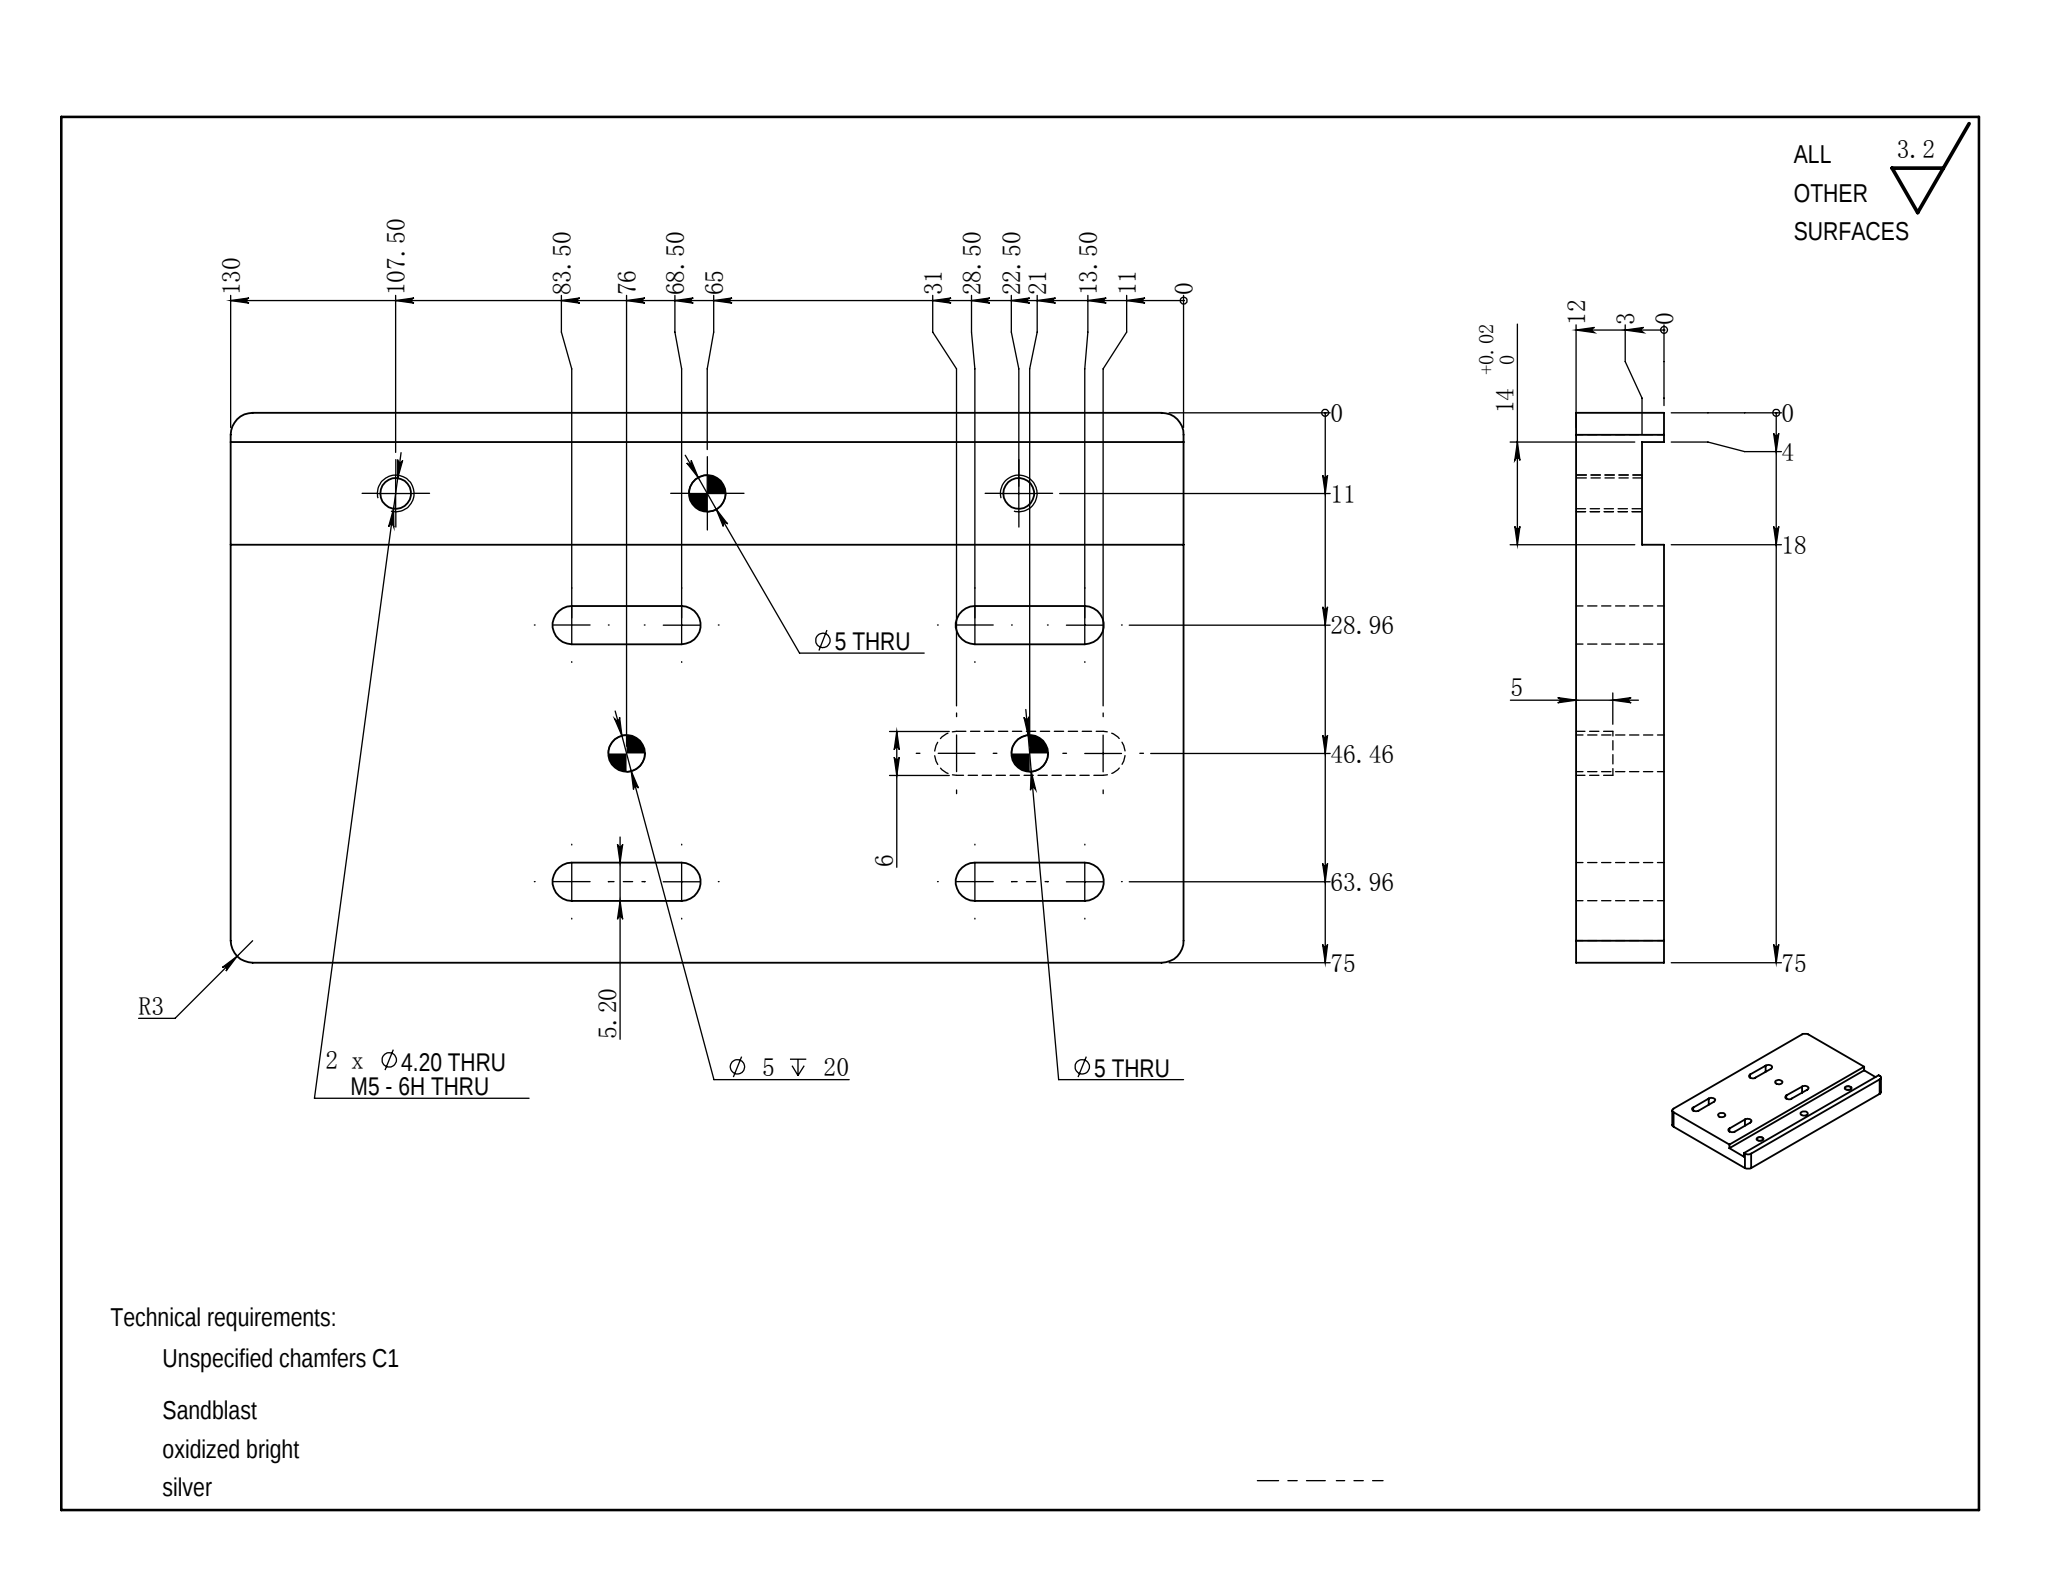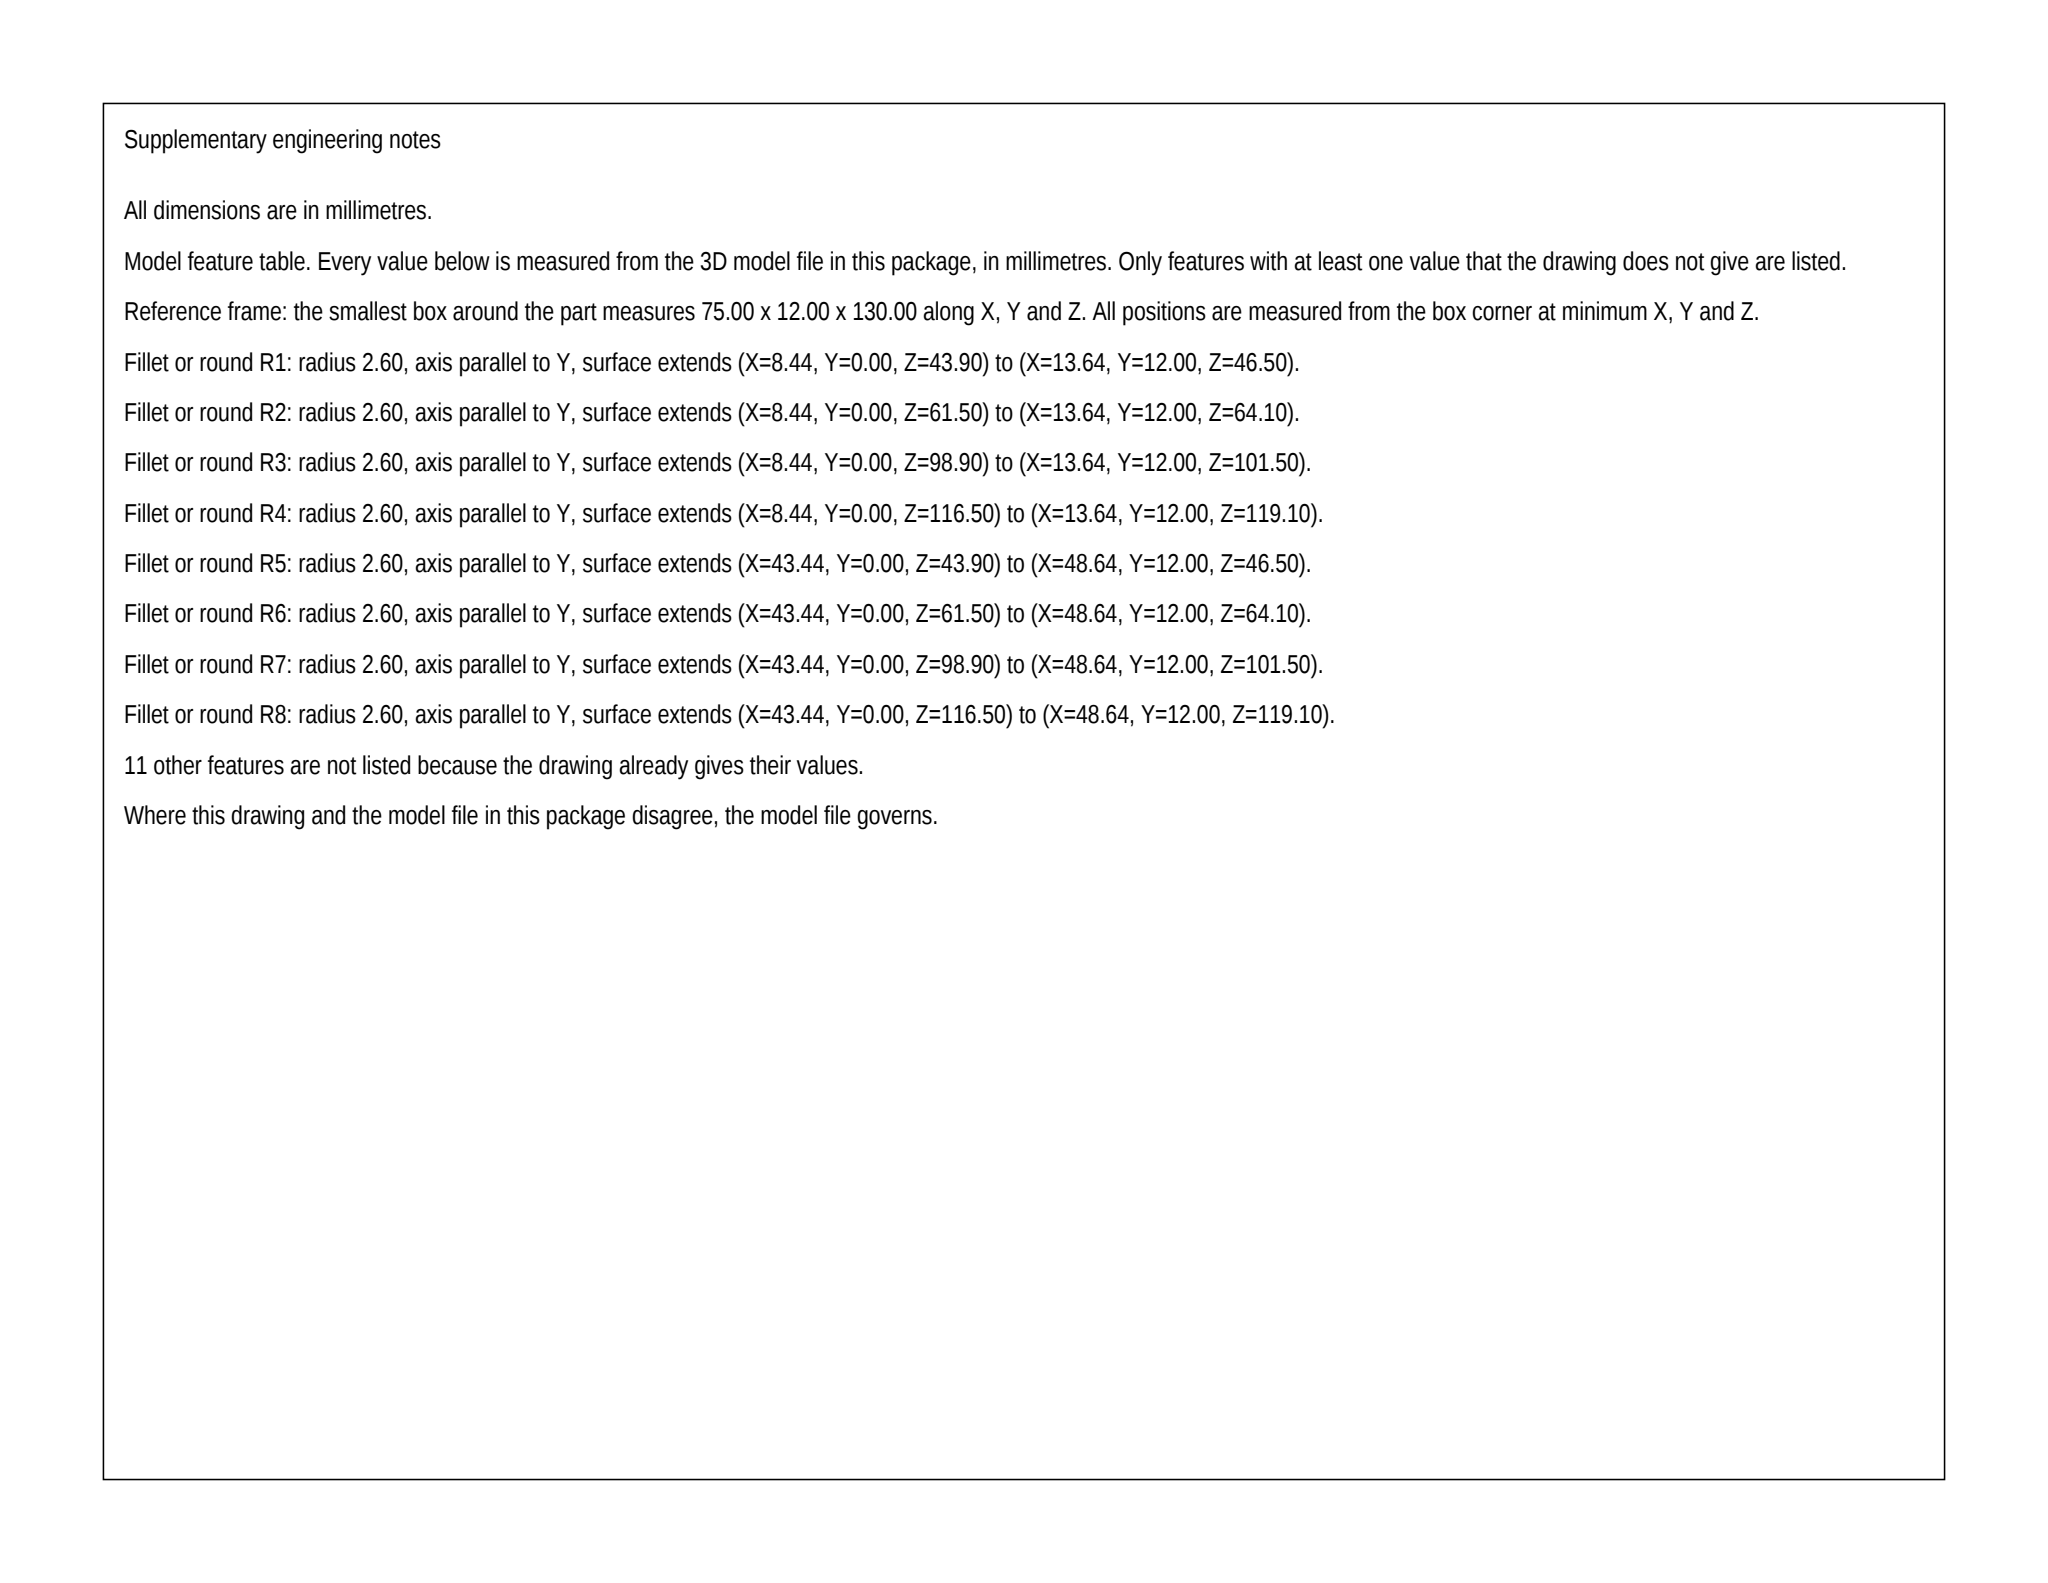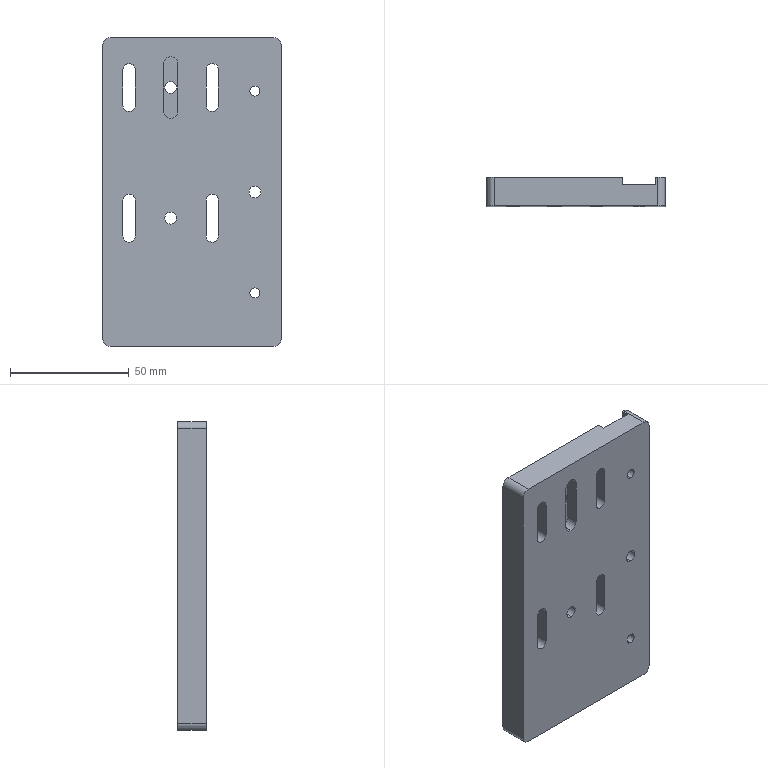Part | SolidWorks | mm | 1 solid | 50 faces | box 75 x 12 x 130 mm | volume 105143 mm3 | cylinder 29 | plane 21 | commonest cylinder face diameters 5.2 x12 6 x7 5 x6 4.2 x4
Drawing notes:
STEP 14 W (4 TO 18) x 3 DP; 9 THK REMAINS | from the solid: x-planes 57 & 71 = Y4/Y18, 14 wide; y-planes 9 & 12 = 3 deep, 9 remaining
4X SLOT 5.20 W x 20.20 LG (15 C-C) THRU 12 | from the solid: Ø5.2 THRU L=12 at x=11.04 & 46.04, z pairs 46.5/61.5 and 101.5/116.5 (15 C-C)
SLOT 6 W x 26 LG (20 C-C) DP 5 W/ Ø5 THRU, CL 46.46 | from the solid: Ø6 L=5 at x=28.54, z=99 & 119 (20 C-C); Ø5 L=7 at x=28.54, z=109; 5+7=12 thk
2X M5 TAP, Ø4.2 DRILL THRU 9 THK, CL 11 AT 22.50 & 107.50 | from the solid: Ø4.2 L=9 at x=64, z=22.5 & 107.5; local thickness 9 at step
Ø5 THRU 9 THK, CL 11 AT 65 | from the solid: Ø5 L=9 at x=64, z=65; local thickness 9 at step
Ø5 THRU 2X AT 46.46 FROM TOP x 76 FROM RIGHT END (NOT ⍋20) | from the solid: cylinder dia 5.0, axis y, pos [28.54, z=54.0], length 12.0 = full 12 plate thickness; 75-28.54=46.46, 130-54=76; count 2
build123d program:
from build123d import *

# Parameters (mm, degrees)
SKETCH1_W                 = 75
SKETCH1_H                 = 130
BOSS_EXTRUDE1_DEPTH       = 12
SKETCH2_W                 = 14
SKETCH2_H                 = 130
CUT_EXTRUDE1_DEPTH        = 3
CUT_EXTRUDE2_DEPTH        = 76.995
LPATTERN1_COUNT           = 2
LPATTERN1_PITCH           = 55
FILLET1_R                 = 3
M5_TAPPED_HOLE1_D         = 4.2
F_5_0_5_DIAMETER_HOLE1_D  = 5
F_5_0_5_DIAMETER_HOLE2_D  = 5
CUT_EXTRUDE3_DEPTH        = 5
SIZE_MM_DOWEL_HOLE1_D     = 5
SIZE_MM_DOWEL_HOLE1_DEPTH = 20
SIZE_MM_DOWEL_HOLE1_TIP   = 1.502


with BuildPart() as part:
    # Sketch1 → Boss-Extrude1 (new body)
    with BuildSketch(Plane(origin=(0, 0, 0), x_dir=(1, 0, 0), z_dir=(0, 1, 0))):
        Rectangle(SKETCH1_W, SKETCH1_H)
    extrude(amount=BOSS_EXTRUDE1_DEPTH)

    # Sketch2 → Cut-Extrude1 (cut)
    with BuildSketch(Plane.XZ.offset(-12)):
        with Locations((26.5, 0)):
            Rectangle(SKETCH2_W, SKETCH2_H)
    extrude(amount=CUT_EXTRUDE1_DEPTH, mode=Mode.SUBTRACT)

    # Sketch3 → Cut-Extrude2 (cut, through all)
    with BuildSketch(Plane(origin=(0, 12, 0), x_dir=(1, 0, 0), z_dir=(0, 1, 0))):
        with BuildLine():
            Line((-29.058, 3.5), (-29.058, 18.5))
            ThreePointArc((-29.058, 18.5), (-26.458, 21.1), (-23.858, 18.5))
            Line((-23.858, 18.5), (-23.858, 3.5))
            ThreePointArc((-23.858, 3.5), (-26.458, 0.9), (-29.058, 3.5))
        make_face()
        with BuildLine():
            Line((11.142, 18.5), (11.142, 3.5))
            ThreePointArc((11.142, 3.5), (8.542, 0.9), (5.942, 3.5))
            Line((5.942, 3.5), (5.942, 18.5))
            ThreePointArc((5.942, 18.5), (8.542, 21.1), (11.142, 18.5))
        make_face()
    cut_extrude2 = extrude(amount=-CUT_EXTRUDE2_DEPTH, mode=Mode.SUBTRACT)

    # LPattern1: Cut-Extrude2 ×2
    with Locations(*[(0, 0, i * LPATTERN1_PITCH) for i in range(1, LPATTERN1_COUNT)]):
        add(cut_extrude2, mode=Mode.SUBTRACT)

    # Fillet1
    fillet1_edges = [part.edges().sort_by_distance(p)[0] for p in [
        (37.5, 6, 65),
        (-37.5, 6, 65),
        (-37.5, 6, -65),
        (37.5, 6, -65),
    ]]
    fillet(fillet1_edges, radius=FILLET1_R)

    # M5 Tapped Hole1 (through all)
    with Locations(Plane(origin=(0, 12, 0), x_dir=(1, 0, 0), z_dir=(0, 1, 0))):
        with Locations((26.5, 42.5), (26.5, -42.5)):
            Hole(M5_TAPPED_HOLE1_D / 2)

    # 5.0 _5_ Diameter Hole1 (through all)
    with Locations(Plane(origin=(0, 9, 0), x_dir=(1, 0, 0), z_dir=(0, 1, 0))):
        with Locations((26.5, 0)):
            Hole(F_5_0_5_DIAMETER_HOLE1_D / 2)

    # 5.0 _5_ Diameter Hole2 (through all)
    with Locations(Plane(origin=(0, 12, 0), x_dir=(1, 0, 0), z_dir=(0, 1, 0))):
        with Locations((-8.958, -44)):
            Hole(F_5_0_5_DIAMETER_HOLE2_D / 2)

    # Sketch15 → Cut-Extrude3 (cut)
    with BuildSketch(Plane.XZ):
        with BuildLine():
            Line((-5.958, 54), (-5.958, 34))
            ThreePointArc((-5.958, 34), (-8.958, 31), (-11.958, 34))
            Line((-11.958, 34), (-11.958, 54))
            ThreePointArc((-11.958, 54), (-8.958, 57), (-5.958, 54))
        make_face()
    extrude(amount=-CUT_EXTRUDE3_DEPTH, mode=Mode.SUBTRACT)

    # Size mm Dowel Hole1
    with Locations(Plane(origin=(-8.958, 12, -11), x_dir=(0, 0, 1), z_dir=(0, 1, 0))):
        with Locations((0, 0)):
            Hole(SIZE_MM_DOWEL_HOLE1_D / 2, depth=SIZE_MM_DOWEL_HOLE1_DEPTH)
            with Locations((0, 0, -(SIZE_MM_DOWEL_HOLE1_DEPTH + SIZE_MM_DOWEL_HOLE1_TIP / 2))):  # 118° drill point
                Cone(0, SIZE_MM_DOWEL_HOLE1_D / 2, SIZE_MM_DOWEL_HOLE1_TIP, mode=Mode.SUBTRACT)


solid = part.part